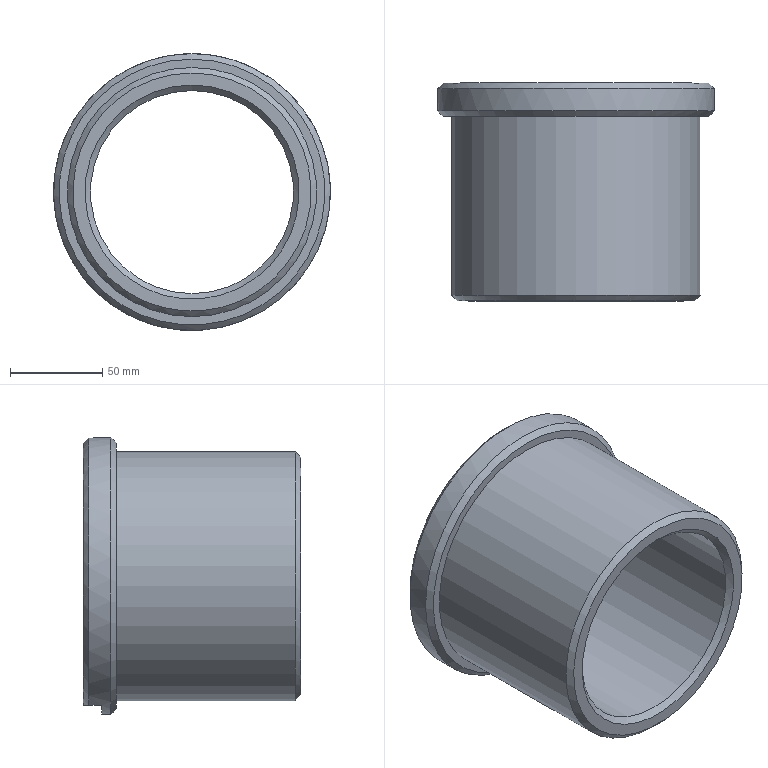Component | NX | BORE_BUSHING | 1 solid | 13 faces | box 150 x 118 x 150 mm | volume 617263 mm3 | plane 5 | cone 5 | cylinder 3 | commonest cylinder face diameters 135 x1 150 x1 110 x1
STEP:
#1=CARTESIAN_POINT('',(0.,0.,0.));
#2=DIRECTION('',(0.,0.,1.));
#3=DIRECTION('',(1.,0.,0.));
#4=AXIS2_PLACEMENT_3D('',#1,#2,#3);
#5=CARTESIAN_POINT('',(0.,42.5,208.));
#6=VERTEX_POINT('',#5);
#7=CARTESIAN_POINT('',(0.,42.5,150.));
#8=DIRECTION('',(0.,1.,0.));
#9=DIRECTION('',(0.,0.,1.));
#10=AXIS2_PLACEMENT_3D('',#7,#8,#9);
#11=CIRCLE('',#10,58.);
#12=CARTESIAN_POINT('',(0.,42.5,150.));
#13=DIRECTION('',(0.,-1.,0.));
#14=DIRECTION('',(0.,0.,1.));
#15=AXIS2_PLACEMENT_3D('',#12,#13,#14);
#16=PLANE('',#15);
#17=CARTESIAN_POINT('',(58.,0.));
#18=CARTESIAN_POINT('',(58.,-100.459));
#19=CARTESIAN_POINT('',(-29.,-50.229));
#20=CARTESIAN_POINT('',(-116.,-0.));
#21=CARTESIAN_POINT('',(-29.,50.229));
#22=CARTESIAN_POINT('',(58.,100.459));
#23=CARTESIAN_POINT('',(58.,0.));
#24=(BOUNDED_CURVE()B_SPLINE_CURVE(2,(#17,#18,#19,#20,#21,#22,#23),.UNSPECIFIED.,.T.,.F.)B_SPLINE_CURVE_WITH_KNOTS((1,2,2,2,2,1),(-2.094,0.,2.094,4.189,6.283,8.378),.UNSPECIFIED.)CURVE()GEOMETRIC_REPRESENTATION_ITEM()RATIONAL_B_SPLINE_CURVE((1.,0.5,1.,0.5,1.,0.5,1.))REPRESENTATION_ITEM(''));
#25=(GEOMETRIC_REPRESENTATION_CONTEXT(2)PARAMETRIC_REPRESENTATION_CONTEXT()REPRESENTATION_CONTEXT('',''));
#26=DEFINITIONAL_REPRESENTATION('',(#24),#25);
#27=PCURVE('',#16,#26);
#28=CARTESIAN_POINT('',(0.,45.5,150.));
#29=DIRECTION('',(0.,-1.,0.));
#30=DIRECTION('',(0.,0.,1.));
#31=AXIS2_PLACEMENT_3D('',#28,#29,#30);
#32=CONICAL_SURFACE('',#31,55.,0.7854);
#33=CARTESIAN_POINT('',(6.283,3.));
#34=DIRECTION('',(-1.,0.));
#35=VECTOR('',#34,1.);
#36=LINE('',#33,#35);
#37=(GEOMETRIC_REPRESENTATION_CONTEXT(2)PARAMETRIC_REPRESENTATION_CONTEXT()REPRESENTATION_CONTEXT('',''));
#38=DEFINITIONAL_REPRESENTATION('',(#36),#37);
#39=PCURVE('',#32,#38);
#40=SURFACE_CURVE('',#11,(#27,#39),.PCURVE_S1.);
#41=EDGE_CURVE('',#6,#6,#40,.T.);
#42=ORIENTED_EDGE('',*,*,#41,.T.);
#43=EDGE_LOOP('',(#42));
#44=FACE_BOUND('',#43,.T.);
#45=CARTESIAN_POINT('',(0.,42.5,214.5));
#46=VERTEX_POINT('',#45);
#47=CARTESIAN_POINT('',(0.,42.5,150.));
#48=DIRECTION('',(0.,-1.,0.));
#49=DIRECTION('',(0.,0.,1.));
#50=AXIS2_PLACEMENT_3D('',#47,#48,#49);
#51=CIRCLE('',#50,64.5);
#52=CARTESIAN_POINT('',(0.,0.));
#53=DIRECTION('',(1.,0.));
#54=AXIS2_PLACEMENT_2D('',#52,#53);
#55=CIRCLE('',#54,64.5);
#56=(GEOMETRIC_REPRESENTATION_CONTEXT(2)PARAMETRIC_REPRESENTATION_CONTEXT()REPRESENTATION_CONTEXT('',''));
#57=DEFINITIONAL_REPRESENTATION('',(#55),#56);
#58=PCURVE('',#16,#57);
#59=CARTESIAN_POINT('',(0.,45.5,150.));
#60=DIRECTION('',(0.,1.,0.));
#61=DIRECTION('',(0.,0.,-1.));
#62=AXIS2_PLACEMENT_3D('',#59,#60,#61);
#63=CONICAL_SURFACE('',#62,67.5,0.7854);
#64=CARTESIAN_POINT('',(9.425,-3.));
#65=DIRECTION('',(-1.,0.));
#66=VECTOR('',#65,1.);
#67=LINE('',#64,#66);
#68=(GEOMETRIC_REPRESENTATION_CONTEXT(2)PARAMETRIC_REPRESENTATION_CONTEXT()REPRESENTATION_CONTEXT('',''));
#69=DEFINITIONAL_REPRESENTATION('',(#67),#68);
#70=PCURVE('',#63,#69);
#71=SURFACE_CURVE('',#51,(#58,#70),.PCURVE_S1.);
#72=EDGE_CURVE('',#46,#46,#71,.T.);
#73=ORIENTED_EDGE('',*,*,#72,.T.);
#74=EDGE_LOOP('',(#73));
#75=FACE_BOUND('',#74,.T.);
#76=ADVANCED_FACE('',(#44,#75),#16,.T.);
#77=CARTESIAN_POINT('',(0.,45.5,217.5));
#78=VERTEX_POINT('',#77);
#79=CARTESIAN_POINT('',(0.,45.5,150.));
#80=DIRECTION('',(0.,1.,0.));
#81=DIRECTION('',(0.,0.,1.));
#82=AXIS2_PLACEMENT_3D('',#79,#80,#81);
#83=CIRCLE('',#82,67.5);
#84=CARTESIAN_POINT('',(0.,42.5,150.));
#85=DIRECTION('',(0.,1.,0.));
#86=DIRECTION('',(0.,0.,-1.));
#87=AXIS2_PLACEMENT_3D('',#84,#85,#86);
#88=CYLINDRICAL_SURFACE('',#87,67.5);
#89=CARTESIAN_POINT('',(3.142,3.));
#90=DIRECTION('',(1.,0.));
#91=VECTOR('',#90,1.);
#92=LINE('',#89,#91);
#93=(GEOMETRIC_REPRESENTATION_CONTEXT(2)PARAMETRIC_REPRESENTATION_CONTEXT()REPRESENTATION_CONTEXT('',''));
#94=DEFINITIONAL_REPRESENTATION('',(#92),#93);
#95=PCURVE('',#88,#94);
#96=CARTESIAN_POINT('',(3.142,0.));
#97=DIRECTION('',(1.,0.));
#98=VECTOR('',#97,1.);
#99=LINE('',#96,#98);
#100=(GEOMETRIC_REPRESENTATION_CONTEXT(2)PARAMETRIC_REPRESENTATION_CONTEXT()REPRESENTATION_CONTEXT('',''));
#101=DEFINITIONAL_REPRESENTATION('',(#99),#100);
#102=PCURVE('',#63,#101);
#103=SURFACE_CURVE('',#83,(#95,#102),.PCURVE_S1.);
#104=EDGE_CURVE('',#78,#78,#103,.T.);
#105=ORIENTED_EDGE('',*,*,#104,.T.);
#106=CARTESIAN_POINT('',(0.,142.5,217.5));
#107=VERTEX_POINT('',#106);
#108=CARTESIAN_POINT('',(-0.,45.5,217.5));
#109=CARTESIAN_POINT('',(-0.,142.5,217.5));
#110=B_SPLINE_CURVE_WITH_KNOTS('',1,(#108,#109),.UNSPECIFIED.,.F.,.F.,(2,2),(3.,100.),.PIECEWISE_BEZIER_KNOTS.);
#111=CARTESIAN_POINT('',(9.425,0.));
#112=DIRECTION('',(0.,1.));
#113=VECTOR('',#112,1.);
#114=LINE('',#111,#113);
#115=(GEOMETRIC_REPRESENTATION_CONTEXT(2)PARAMETRIC_REPRESENTATION_CONTEXT()REPRESENTATION_CONTEXT('',''));
#116=DEFINITIONAL_REPRESENTATION('',(#114),#115);
#117=PCURVE('',#88,#116);
#118=CARTESIAN_POINT('',(3.142,0.));
#119=DIRECTION('',(0.,1.));
#120=VECTOR('',#119,1.);
#121=LINE('',#118,#120);
#122=(GEOMETRIC_REPRESENTATION_CONTEXT(2)PARAMETRIC_REPRESENTATION_CONTEXT()REPRESENTATION_CONTEXT('',''));
#123=DEFINITIONAL_REPRESENTATION('',(#121),#122);
#124=PCURVE('',#88,#123);
#125=SEAM_CURVE('',#110,(#117,#124),.PCURVE_S1.);
#126=EDGE_CURVE('',#78,#107,#125,.T.);
#127=ORIENTED_EDGE('',*,*,#126,.T.);
#128=CARTESIAN_POINT('',(0.,142.5,150.));
#129=DIRECTION('',(0.,1.,0.));
#130=DIRECTION('',(0.,0.,1.));
#131=AXIS2_PLACEMENT_3D('',#128,#129,#130);
#132=CIRCLE('',#131,67.5);
#133=CARTESIAN_POINT('',(3.142,100.));
#134=DIRECTION('',(1.,0.));
#135=VECTOR('',#134,1.);
#136=LINE('',#133,#135);
#137=(GEOMETRIC_REPRESENTATION_CONTEXT(2)PARAMETRIC_REPRESENTATION_CONTEXT()REPRESENTATION_CONTEXT('',''));
#138=DEFINITIONAL_REPRESENTATION('',(#136),#137);
#139=PCURVE('',#88,#138);
#140=CARTESIAN_POINT('',(0.,142.5,150.));
#141=DIRECTION('',(0.,-1.,0.));
#142=DIRECTION('',(0.,0.,1.));
#143=AXIS2_PLACEMENT_3D('',#140,#141,#142);
#144=PLANE('',#143);
#145=CARTESIAN_POINT('',(67.5,0.));
#146=CARTESIAN_POINT('',(67.5,-116.913));
#147=CARTESIAN_POINT('',(-33.75,-58.457));
#148=CARTESIAN_POINT('',(-135.,-0.));
#149=CARTESIAN_POINT('',(-33.75,58.457));
#150=CARTESIAN_POINT('',(67.5,116.913));
#151=CARTESIAN_POINT('',(67.5,0.));
#152=(BOUNDED_CURVE()B_SPLINE_CURVE(2,(#145,#146,#147,#148,#149,#150,#151),.UNSPECIFIED.,.T.,.F.)B_SPLINE_CURVE_WITH_KNOTS((1,2,2,2,2,1),(-2.094,0.,2.094,4.189,6.283,8.378),.UNSPECIFIED.)CURVE()GEOMETRIC_REPRESENTATION_ITEM()RATIONAL_B_SPLINE_CURVE((1.,0.5,1.,0.5,1.,0.5,1.))REPRESENTATION_ITEM(''));
#153=(GEOMETRIC_REPRESENTATION_CONTEXT(2)PARAMETRIC_REPRESENTATION_CONTEXT()REPRESENTATION_CONTEXT('',''));
#154=DEFINITIONAL_REPRESENTATION('',(#152),#153);
#155=PCURVE('',#144,#154);
#156=SURFACE_CURVE('',#132,(#139,#155),.PCURVE_S1.);
#157=EDGE_CURVE('',#107,#107,#156,.T.);
#158=ORIENTED_EDGE('',*,*,#157,.F.);
#159=ORIENTED_EDGE('',*,*,#126,.F.);
#160=EDGE_LOOP('',(#105,#127,#158,#159));
#161=FACE_BOUND('',#160,.T.);
#162=ADVANCED_FACE('',(#161),#88,.T.);
#163=CARTESIAN_POINT('',(0.,160.5,92.));
#164=VERTEX_POINT('',#163);
#165=CARTESIAN_POINT('',(0.,160.5,150.));
#166=DIRECTION('',(0.,-1.,0.));
#167=DIRECTION('',(0.,0.,-1.));
#168=AXIS2_PLACEMENT_3D('',#165,#166,#167);
#169=CIRCLE('',#168,58.);
#170=CARTESIAN_POINT('',(0.,160.5,150.));
#171=DIRECTION('',(0.,1.,0.));
#172=DIRECTION('',(0.,0.,-1.));
#173=AXIS2_PLACEMENT_3D('',#170,#171,#172);
#174=PLANE('',#173);
#175=CARTESIAN_POINT('',(58.,0.));
#176=CARTESIAN_POINT('',(58.,-100.459));
#177=CARTESIAN_POINT('',(-29.,-50.229));
#178=CARTESIAN_POINT('',(-116.,-0.));
#179=CARTESIAN_POINT('',(-29.,50.229));
#180=CARTESIAN_POINT('',(58.,100.459));
#181=CARTESIAN_POINT('',(58.,0.));
#182=(BOUNDED_CURVE()B_SPLINE_CURVE(2,(#175,#176,#177,#178,#179,#180,#181),.UNSPECIFIED.,.T.,.F.)B_SPLINE_CURVE_WITH_KNOTS((1,2,2,2,2,1),(-2.094,0.,2.094,4.189,6.283,8.378),.UNSPECIFIED.)CURVE()GEOMETRIC_REPRESENTATION_ITEM()RATIONAL_B_SPLINE_CURVE((1.,0.5,1.,0.5,1.,0.5,1.))REPRESENTATION_ITEM(''));
#183=(GEOMETRIC_REPRESENTATION_CONTEXT(2)PARAMETRIC_REPRESENTATION_CONTEXT()REPRESENTATION_CONTEXT('',''));
#184=DEFINITIONAL_REPRESENTATION('',(#182),#183);
#185=PCURVE('',#174,#184);
#186=CARTESIAN_POINT('',(0.,160.5,150.));
#187=DIRECTION('',(0.,1.,0.));
#188=DIRECTION('',(0.,0.,-1.));
#189=AXIS2_PLACEMENT_3D('',#186,#187,#188);
#190=CONICAL_SURFACE('',#189,58.,0.7854);
#191=CARTESIAN_POINT('',(6.283,0.));
#192=DIRECTION('',(-1.,0.));
#193=VECTOR('',#192,1.);
#194=LINE('',#191,#193);
#195=(GEOMETRIC_REPRESENTATION_CONTEXT(2)PARAMETRIC_REPRESENTATION_CONTEXT()REPRESENTATION_CONTEXT('',''));
#196=DEFINITIONAL_REPRESENTATION('',(#194),#195);
#197=PCURVE('',#190,#196);
#198=SURFACE_CURVE('',#169,(#185,#197),.PCURVE_S1.);
#199=EDGE_CURVE('',#164,#164,#198,.T.);
#200=ORIENTED_EDGE('',*,*,#199,.T.);
#201=EDGE_LOOP('',(#200));
#202=FACE_BOUND('',#201,.T.);
#203=CARTESIAN_POINT('',(-16.852,160.5,80.));
#204=VERTEX_POINT('',#203);
#205=CARTESIAN_POINT('',(16.852,160.5,80.));
#206=VERTEX_POINT('',#205);
#207=CARTESIAN_POINT('',(-76.,160.5,80.));
#208=DIRECTION('',(1.,0.,-0.));
#209=VECTOR('',#208,1.);
#210=LINE('',#207,#209);
#211=CARTESIAN_POINT('',(70.,76.));
#212=DIRECTION('',(0.,-1.));
#213=VECTOR('',#212,1.);
#214=LINE('',#211,#213);
#215=(GEOMETRIC_REPRESENTATION_CONTEXT(2)PARAMETRIC_REPRESENTATION_CONTEXT()REPRESENTATION_CONTEXT('',''));
#216=DEFINITIONAL_REPRESENTATION('',(#214),#215);
#217=PCURVE('',#174,#216);
#218=CARTESIAN_POINT('',(-76.,150.5,80.));
#219=DIRECTION('',(0.,0.,1.));
#220=DIRECTION('',(1.,0.,-0.));
#221=AXIS2_PLACEMENT_3D('',#218,#219,#220);
#222=PLANE('',#221);
#223=CARTESIAN_POINT('',(0.,10.));
#224=DIRECTION('',(1.,0.));
#225=VECTOR('',#224,1.);
#226=LINE('',#223,#225);
#227=(GEOMETRIC_REPRESENTATION_CONTEXT(2)PARAMETRIC_REPRESENTATION_CONTEXT()REPRESENTATION_CONTEXT('',''));
#228=DEFINITIONAL_REPRESENTATION('',(#226),#227);
#229=PCURVE('',#222,#228);
#230=SURFACE_CURVE('',#210,(#217,#229),.PCURVE_S1.);
#231=EDGE_CURVE('',#204,#206,#230,.T.);
#232=ORIENTED_EDGE('',*,*,#231,.F.);
#233=CARTESIAN_POINT('',(0.,160.5,150.));
#234=DIRECTION('',(0.,1.,0.));
#235=DIRECTION('',(0.,0.,-1.));
#236=AXIS2_PLACEMENT_3D('',#233,#234,#235);
#237=CIRCLE('',#236,72.);
#238=CARTESIAN_POINT('',(0.,0.));
#239=DIRECTION('',(1.,0.));
#240=AXIS2_PLACEMENT_2D('',#238,#239);
#241=CIRCLE('',#240,72.);
#242=(GEOMETRIC_REPRESENTATION_CONTEXT(2)PARAMETRIC_REPRESENTATION_CONTEXT()REPRESENTATION_CONTEXT('',''));
#243=DEFINITIONAL_REPRESENTATION('',(#241),#242);
#244=PCURVE('',#174,#243);
#245=CARTESIAN_POINT('',(0.,157.5,150.));
#246=DIRECTION('',(0.,-1.,0.));
#247=DIRECTION('',(0.,0.,1.));
#248=AXIS2_PLACEMENT_3D('',#245,#246,#247);
#249=CONICAL_SURFACE('',#248,75.,0.7854);
#250=CARTESIAN_POINT('',(3.142,-3.));
#251=DIRECTION('',(-1.,0.));
#252=VECTOR('',#251,1.);
#253=LINE('',#250,#252);
#254=(GEOMETRIC_REPRESENTATION_CONTEXT(2)PARAMETRIC_REPRESENTATION_CONTEXT()REPRESENTATION_CONTEXT('',''));
#255=DEFINITIONAL_REPRESENTATION('',(#253),#254);
#256=PCURVE('',#249,#255);
#257=SURFACE_CURVE('',#237,(#244,#256),.PCURVE_S1.);
#258=EDGE_CURVE('',#204,#206,#257,.T.);
#259=ORIENTED_EDGE('',*,*,#258,.T.);
#260=EDGE_LOOP('',(#232,#259));
#261=FACE_BOUND('',#260,.T.);
#262=ADVANCED_FACE('',(#202,#261),#174,.T.);
#263=CARTESIAN_POINT('',(0.,142.5,222.));
#264=VERTEX_POINT('',#263);
#265=CARTESIAN_POINT('',(0.,142.5,150.));
#266=DIRECTION('',(0.,-1.,0.));
#267=DIRECTION('',(0.,0.,1.));
#268=AXIS2_PLACEMENT_3D('',#265,#266,#267);
#269=CIRCLE('',#268,72.);
#270=CARTESIAN_POINT('',(0.,0.));
#271=DIRECTION('',(1.,0.));
#272=AXIS2_PLACEMENT_2D('',#270,#271);
#273=CIRCLE('',#272,72.);
#274=(GEOMETRIC_REPRESENTATION_CONTEXT(2)PARAMETRIC_REPRESENTATION_CONTEXT()REPRESENTATION_CONTEXT('',''));
#275=DEFINITIONAL_REPRESENTATION('',(#273),#274);
#276=PCURVE('',#144,#275);
#277=CARTESIAN_POINT('',(0.,145.5,150.));
#278=DIRECTION('',(0.,1.,0.));
#279=DIRECTION('',(0.,0.,-1.));
#280=AXIS2_PLACEMENT_3D('',#277,#278,#279);
#281=CONICAL_SURFACE('',#280,75.,0.7854);
#282=CARTESIAN_POINT('',(9.425,-3.));
#283=DIRECTION('',(-1.,0.));
#284=VECTOR('',#283,1.);
#285=LINE('',#282,#284);
#286=(GEOMETRIC_REPRESENTATION_CONTEXT(2)PARAMETRIC_REPRESENTATION_CONTEXT()REPRESENTATION_CONTEXT('',''));
#287=DEFINITIONAL_REPRESENTATION('',(#285),#286);
#288=PCURVE('',#281,#287);
#289=SURFACE_CURVE('',#269,(#276,#288),.PCURVE_S1.);
#290=EDGE_CURVE('',#264,#264,#289,.T.);
#291=ORIENTED_EDGE('',*,*,#290,.T.);
#292=EDGE_LOOP('',(#291));
#293=FACE_BOUND('',#292,.T.);
#294=ORIENTED_EDGE('',*,*,#157,.T.);
#295=EDGE_LOOP('',(#294));
#296=FACE_BOUND('',#295,.T.);
#297=ADVANCED_FACE('',(#293,#296),#144,.T.);
#298=CARTESIAN_POINT('',(0.,145.5,225.));
#299=VERTEX_POINT('',#298);
#300=CARTESIAN_POINT('',(26.926,145.5,80.));
#301=VERTEX_POINT('',#300);
#302=CARTESIAN_POINT('',(0.,145.5,150.));
#303=DIRECTION('',(0.,1.,0.));
#304=DIRECTION('',(0.,0.,1.));
#305=AXIS2_PLACEMENT_3D('',#302,#303,#304);
#306=CIRCLE('',#305,75.);
#307=CARTESIAN_POINT('',(0.,142.5,150.));
#308=DIRECTION('',(0.,1.,0.));
#309=DIRECTION('',(0.,0.,-1.));
#310=AXIS2_PLACEMENT_3D('',#307,#308,#309);
#311=CYLINDRICAL_SURFACE('',#310,75.);
#312=CARTESIAN_POINT('',(9.425,3.));
#313=DIRECTION('',(1.,0.));
#314=VECTOR('',#313,1.);
#315=LINE('',#312,#314);
#316=(GEOMETRIC_REPRESENTATION_CONTEXT(2)PARAMETRIC_REPRESENTATION_CONTEXT()REPRESENTATION_CONTEXT('',''));
#317=DEFINITIONAL_REPRESENTATION('',(#315),#316);
#318=PCURVE('',#311,#317);
#319=CARTESIAN_POINT('',(3.142,0.));
#320=DIRECTION('',(1.,0.));
#321=VECTOR('',#320,1.);
#322=LINE('',#319,#321);
#323=(GEOMETRIC_REPRESENTATION_CONTEXT(2)PARAMETRIC_REPRESENTATION_CONTEXT()REPRESENTATION_CONTEXT('',''));
#324=DEFINITIONAL_REPRESENTATION('',(#322),#323);
#325=PCURVE('',#281,#324);
#326=SURFACE_CURVE('',#306,(#318,#325),.PCURVE_S1.);
#327=EDGE_CURVE('',#299,#301,#326,.T.);
#328=ORIENTED_EDGE('',*,*,#327,.T.);
#329=CARTESIAN_POINT('',(26.926,150.5,80.));
#330=VERTEX_POINT('',#329);
#331=CARTESIAN_POINT('',(26.926,145.5,80.));
#332=CARTESIAN_POINT('',(26.926,150.5,80.));
#333=B_SPLINE_CURVE_WITH_KNOTS('',1,(#331,#332),.UNSPECIFIED.,.F.,.F.,(2,2),(3.,8.),.PIECEWISE_BEZIER_KNOTS.);
#334=CARTESIAN_POINT('',(12.199,0.));
#335=DIRECTION('',(0.,1.));
#336=VECTOR('',#335,1.);
#337=LINE('',#334,#336);
#338=(GEOMETRIC_REPRESENTATION_CONTEXT(2)PARAMETRIC_REPRESENTATION_CONTEXT()REPRESENTATION_CONTEXT('',''));
#339=DEFINITIONAL_REPRESENTATION('',(#337),#338);
#340=PCURVE('',#311,#339);
#341=CARTESIAN_POINT('',(5.916,0.));
#342=DIRECTION('',(0.,1.));
#343=VECTOR('',#342,1.);
#344=LINE('',#341,#343);
#345=(GEOMETRIC_REPRESENTATION_CONTEXT(2)PARAMETRIC_REPRESENTATION_CONTEXT()REPRESENTATION_CONTEXT('',''));
#346=DEFINITIONAL_REPRESENTATION('',(#344),#345);
#347=PCURVE('',#311,#346);
#348=SEAM_CURVE('',#333,(#340,#347),.PCURVE_S1.);
#349=EDGE_CURVE('',#301,#330,#348,.T.);
#350=ORIENTED_EDGE('',*,*,#349,.T.);
#351=CARTESIAN_POINT('',(26.926,157.5,80.));
#352=VERTEX_POINT('',#351);
#353=CARTESIAN_POINT('',(26.926,142.5,80.));
#354=DIRECTION('',(0.,-1.,0.));
#355=VECTOR('',#354,1.);
#356=LINE('',#353,#355);
#357=CARTESIAN_POINT('',(12.199,0.));
#358=DIRECTION('',(0.,-1.));
#359=VECTOR('',#358,1.);
#360=LINE('',#357,#359);
#361=(GEOMETRIC_REPRESENTATION_CONTEXT(2)PARAMETRIC_REPRESENTATION_CONTEXT()REPRESENTATION_CONTEXT('',''));
#362=DEFINITIONAL_REPRESENTATION('',(#360),#361);
#363=PCURVE('',#311,#362);
#364=CARTESIAN_POINT('',(102.926,-8.));
#365=DIRECTION('',(0.,-1.));
#366=VECTOR('',#365,1.);
#367=LINE('',#364,#366);
#368=(GEOMETRIC_REPRESENTATION_CONTEXT(2)PARAMETRIC_REPRESENTATION_CONTEXT()REPRESENTATION_CONTEXT('',''));
#369=DEFINITIONAL_REPRESENTATION('',(#367),#368);
#370=PCURVE('',#222,#369);
#371=SURFACE_CURVE('',#356,(#363,#370),.PCURVE_S1.);
#372=EDGE_CURVE('',#352,#330,#371,.T.);
#373=ORIENTED_EDGE('',*,*,#372,.F.);
#374=CARTESIAN_POINT('',(-26.926,157.5,80.));
#375=VERTEX_POINT('',#374);
#376=CARTESIAN_POINT('',(0.,157.5,150.));
#377=DIRECTION('',(0.,-1.,0.));
#378=DIRECTION('',(0.,0.,-1.));
#379=AXIS2_PLACEMENT_3D('',#376,#377,#378);
#380=CIRCLE('',#379,75.);
#381=CARTESIAN_POINT('',(12.566,15.));
#382=DIRECTION('',(-1.,0.));
#383=VECTOR('',#382,1.);
#384=LINE('',#381,#383);
#385=(GEOMETRIC_REPRESENTATION_CONTEXT(2)PARAMETRIC_REPRESENTATION_CONTEXT()REPRESENTATION_CONTEXT('',''));
#386=DEFINITIONAL_REPRESENTATION('',(#384),#385);
#387=PCURVE('',#311,#386);
#388=CARTESIAN_POINT('',(-3.142,0.));
#389=DIRECTION('',(1.,0.));
#390=VECTOR('',#389,1.);
#391=LINE('',#388,#390);
#392=(GEOMETRIC_REPRESENTATION_CONTEXT(2)PARAMETRIC_REPRESENTATION_CONTEXT()REPRESENTATION_CONTEXT('',''));
#393=DEFINITIONAL_REPRESENTATION('',(#391),#392);
#394=PCURVE('',#249,#393);
#395=SURFACE_CURVE('',#380,(#387,#394),.PCURVE_S1.);
#396=EDGE_CURVE('',#352,#375,#395,.T.);
#397=ORIENTED_EDGE('',*,*,#396,.T.);
#398=CARTESIAN_POINT('',(-26.926,150.5,80.));
#399=VERTEX_POINT('',#398);
#400=CARTESIAN_POINT('',(-26.926,142.5,80.));
#401=DIRECTION('',(0.,1.,0.));
#402=VECTOR('',#401,1.);
#403=LINE('',#400,#402);
#404=CARTESIAN_POINT('',(6.65,0.));
#405=DIRECTION('',(0.,1.));
#406=VECTOR('',#405,1.);
#407=LINE('',#404,#406);
#408=(GEOMETRIC_REPRESENTATION_CONTEXT(2)PARAMETRIC_REPRESENTATION_CONTEXT()REPRESENTATION_CONTEXT('',''));
#409=DEFINITIONAL_REPRESENTATION('',(#407),#408);
#410=PCURVE('',#311,#409);
#411=CARTESIAN_POINT('',(49.074,-8.));
#412=DIRECTION('',(0.,1.));
#413=VECTOR('',#412,1.);
#414=LINE('',#411,#413);
#415=(GEOMETRIC_REPRESENTATION_CONTEXT(2)PARAMETRIC_REPRESENTATION_CONTEXT()REPRESENTATION_CONTEXT('',''));
#416=DEFINITIONAL_REPRESENTATION('',(#414),#415);
#417=PCURVE('',#222,#416);
#418=SURFACE_CURVE('',#403,(#410,#417),.PCURVE_S1.);
#419=EDGE_CURVE('',#399,#375,#418,.T.);
#420=ORIENTED_EDGE('',*,*,#419,.F.);
#421=CARTESIAN_POINT('',(0.,150.5,150.));
#422=DIRECTION('',(0.,-1.,0.));
#423=DIRECTION('',(0.,0.,-1.));
#424=AXIS2_PLACEMENT_3D('',#421,#422,#423);
#425=CIRCLE('',#424,75.);
#426=CARTESIAN_POINT('',(12.566,8.));
#427=DIRECTION('',(-1.,0.));
#428=VECTOR('',#427,1.);
#429=LINE('',#426,#428);
#430=(GEOMETRIC_REPRESENTATION_CONTEXT(2)PARAMETRIC_REPRESENTATION_CONTEXT()REPRESENTATION_CONTEXT('',''));
#431=DEFINITIONAL_REPRESENTATION('',(#429),#430);
#432=PCURVE('',#311,#431);
#433=CARTESIAN_POINT('',(0.,150.5,150.));
#434=DIRECTION('',(0.,1.,0.));
#435=DIRECTION('',(0.,0.,-1.));
#436=AXIS2_PLACEMENT_3D('',#433,#434,#435);
#437=PLANE('',#436);
#438=CARTESIAN_POINT('',(75.,0.));
#439=CARTESIAN_POINT('',(75.,-129.904));
#440=CARTESIAN_POINT('',(-37.5,-64.952));
#441=CARTESIAN_POINT('',(-150.,-0.));
#442=CARTESIAN_POINT('',(-37.5,64.952));
#443=CARTESIAN_POINT('',(75.,129.904));
#444=CARTESIAN_POINT('',(75.,0.));
#445=(BOUNDED_CURVE()B_SPLINE_CURVE(2,(#438,#439,#440,#441,#442,#443,#444),.UNSPECIFIED.,.T.,.F.)B_SPLINE_CURVE_WITH_KNOTS((1,2,2,2,2,1),(-2.094,0.,2.094,4.189,6.283,8.378),.UNSPECIFIED.)CURVE()GEOMETRIC_REPRESENTATION_ITEM()RATIONAL_B_SPLINE_CURVE((1.,0.5,1.,0.5,1.,0.5,1.))REPRESENTATION_ITEM(''));
#446=(GEOMETRIC_REPRESENTATION_CONTEXT(2)PARAMETRIC_REPRESENTATION_CONTEXT()REPRESENTATION_CONTEXT('',''));
#447=DEFINITIONAL_REPRESENTATION('',(#445),#446);
#448=PCURVE('',#437,#447);
#449=SURFACE_CURVE('',#425,(#432,#448),.PCURVE_S1.);
#450=EDGE_CURVE('',#399,#330,#449,.T.);
#451=ORIENTED_EDGE('',*,*,#450,.T.);
#452=ORIENTED_EDGE('',*,*,#349,.F.);
#453=CARTESIAN_POINT('',(0.,145.5,150.));
#454=DIRECTION('',(0.,1.,0.));
#455=DIRECTION('',(0.,0.,1.));
#456=AXIS2_PLACEMENT_3D('',#453,#454,#455);
#457=CIRCLE('',#456,75.);
#458=CARTESIAN_POINT('',(3.142,3.));
#459=DIRECTION('',(1.,0.));
#460=VECTOR('',#459,1.);
#461=LINE('',#458,#460);
#462=(GEOMETRIC_REPRESENTATION_CONTEXT(2)PARAMETRIC_REPRESENTATION_CONTEXT()REPRESENTATION_CONTEXT('',''));
#463=DEFINITIONAL_REPRESENTATION('',(#461),#462);
#464=PCURVE('',#311,#463);
#465=CARTESIAN_POINT('',(3.142,0.));
#466=DIRECTION('',(1.,0.));
#467=VECTOR('',#466,1.);
#468=LINE('',#465,#467);
#469=(GEOMETRIC_REPRESENTATION_CONTEXT(2)PARAMETRIC_REPRESENTATION_CONTEXT()REPRESENTATION_CONTEXT('',''));
#470=DEFINITIONAL_REPRESENTATION('',(#468),#469);
#471=PCURVE('',#281,#470);
#472=SURFACE_CURVE('',#457,(#464,#471),.PCURVE_S1.);
#473=EDGE_CURVE('',#301,#299,#472,.T.);
#474=ORIENTED_EDGE('',*,*,#473,.T.);
#475=EDGE_LOOP('',(#328,#350,#373,#397,#420,#451,#452,#474));
#476=FACE_BOUND('',#475,.T.);
#477=ADVANCED_FACE('',(#476),#311,.T.);
#478=CARTESIAN_POINT('',(0.,45.5,205.));
#479=VERTEX_POINT('',#478);
#480=CARTESIAN_POINT('',(0.,45.5,150.));
#481=DIRECTION('',(0.,-1.,0.));
#482=DIRECTION('',(0.,0.,1.));
#483=AXIS2_PLACEMENT_3D('',#480,#481,#482);
#484=CIRCLE('',#483,55.);
#485=CARTESIAN_POINT('',(0.,160.5,150.));
#486=DIRECTION('',(0.,-1.,0.));
#487=DIRECTION('',(0.,0.,1.));
#488=AXIS2_PLACEMENT_3D('',#485,#486,#487);
#489=CYLINDRICAL_SURFACE('',#488,55.);
#490=CARTESIAN_POINT('',(0.,115.));
#491=DIRECTION('',(1.,0.));
#492=VECTOR('',#491,1.);
#493=LINE('',#490,#492);
#494=(GEOMETRIC_REPRESENTATION_CONTEXT(2)PARAMETRIC_REPRESENTATION_CONTEXT()REPRESENTATION_CONTEXT('',''));
#495=DEFINITIONAL_REPRESENTATION('',(#493),#494);
#496=PCURVE('',#489,#495);
#497=CARTESIAN_POINT('',(0.,0.));
#498=DIRECTION('',(1.,0.));
#499=VECTOR('',#498,1.);
#500=LINE('',#497,#499);
#501=(GEOMETRIC_REPRESENTATION_CONTEXT(2)PARAMETRIC_REPRESENTATION_CONTEXT()REPRESENTATION_CONTEXT('',''));
#502=DEFINITIONAL_REPRESENTATION('',(#500),#501);
#503=PCURVE('',#32,#502);
#504=SURFACE_CURVE('',#484,(#496,#503),.PCURVE_S1.);
#505=EDGE_CURVE('',#479,#479,#504,.T.);
#506=ORIENTED_EDGE('',*,*,#505,.F.);
#507=CARTESIAN_POINT('',(0.,157.5,205.));
#508=VERTEX_POINT('',#507);
#509=CARTESIAN_POINT('',(0.,157.5,205.));
#510=CARTESIAN_POINT('',(0.,45.5,205.));
#511=B_SPLINE_CURVE_WITH_KNOTS('',1,(#509,#510),.UNSPECIFIED.,.F.,.F.,(2,2),(3.,115.),.PIECEWISE_BEZIER_KNOTS.);
#512=CARTESIAN_POINT('',(0.,0.));
#513=DIRECTION('',(0.,1.));
#514=VECTOR('',#513,1.);
#515=LINE('',#512,#514);
#516=(GEOMETRIC_REPRESENTATION_CONTEXT(2)PARAMETRIC_REPRESENTATION_CONTEXT()REPRESENTATION_CONTEXT('',''));
#517=DEFINITIONAL_REPRESENTATION('',(#515),#516);
#518=PCURVE('',#489,#517);
#519=CARTESIAN_POINT('',(6.283,0.));
#520=DIRECTION('',(0.,1.));
#521=VECTOR('',#520,1.);
#522=LINE('',#519,#521);
#523=(GEOMETRIC_REPRESENTATION_CONTEXT(2)PARAMETRIC_REPRESENTATION_CONTEXT()REPRESENTATION_CONTEXT('',''));
#524=DEFINITIONAL_REPRESENTATION('',(#522),#523);
#525=PCURVE('',#489,#524);
#526=SEAM_CURVE('',#511,(#518,#525),.PCURVE_S1.);
#527=EDGE_CURVE('',#508,#479,#526,.T.);
#528=ORIENTED_EDGE('',*,*,#527,.F.);
#529=CARTESIAN_POINT('',(0.,157.5,95.));
#530=VERTEX_POINT('',#529);
#531=CARTESIAN_POINT('',(0.,157.5,150.));
#532=DIRECTION('',(0.,1.,0.));
#533=DIRECTION('',(0.,0.,-1.));
#534=AXIS2_PLACEMENT_3D('',#531,#532,#533);
#535=CIRCLE('',#534,55.);
#536=CARTESIAN_POINT('',(3.142,3.));
#537=DIRECTION('',(-1.,0.));
#538=VECTOR('',#537,1.);
#539=LINE('',#536,#538);
#540=(GEOMETRIC_REPRESENTATION_CONTEXT(2)PARAMETRIC_REPRESENTATION_CONTEXT()REPRESENTATION_CONTEXT('',''));
#541=DEFINITIONAL_REPRESENTATION('',(#539),#540);
#542=PCURVE('',#489,#541);
#543=CARTESIAN_POINT('',(0.,-3.));
#544=DIRECTION('',(1.,0.));
#545=VECTOR('',#544,1.);
#546=LINE('',#543,#545);
#547=(GEOMETRIC_REPRESENTATION_CONTEXT(2)PARAMETRIC_REPRESENTATION_CONTEXT()REPRESENTATION_CONTEXT('',''));
#548=DEFINITIONAL_REPRESENTATION('',(#546),#547);
#549=PCURVE('',#190,#548);
#550=SURFACE_CURVE('',#535,(#542,#549),.PCURVE_S1.);
#551=EDGE_CURVE('',#530,#508,#550,.T.);
#552=ORIENTED_EDGE('',*,*,#551,.F.);
#553=CARTESIAN_POINT('',(0.,157.5,150.));
#554=DIRECTION('',(0.,1.,0.));
#555=DIRECTION('',(0.,0.,-1.));
#556=AXIS2_PLACEMENT_3D('',#553,#554,#555);
#557=CIRCLE('',#556,55.);
#558=CARTESIAN_POINT('',(9.425,3.));
#559=DIRECTION('',(-1.,0.));
#560=VECTOR('',#559,1.);
#561=LINE('',#558,#560);
#562=(GEOMETRIC_REPRESENTATION_CONTEXT(2)PARAMETRIC_REPRESENTATION_CONTEXT()REPRESENTATION_CONTEXT('',''));
#563=DEFINITIONAL_REPRESENTATION('',(#561),#562);
#564=PCURVE('',#489,#563);
#565=CARTESIAN_POINT('',(0.,-3.));
#566=DIRECTION('',(1.,0.));
#567=VECTOR('',#566,1.);
#568=LINE('',#565,#567);
#569=(GEOMETRIC_REPRESENTATION_CONTEXT(2)PARAMETRIC_REPRESENTATION_CONTEXT()REPRESENTATION_CONTEXT('',''));
#570=DEFINITIONAL_REPRESENTATION('',(#568),#569);
#571=PCURVE('',#190,#570);
#572=SURFACE_CURVE('',#557,(#564,#571),.PCURVE_S1.);
#573=EDGE_CURVE('',#508,#530,#572,.T.);
#574=ORIENTED_EDGE('',*,*,#573,.F.);
#575=ORIENTED_EDGE('',*,*,#527,.T.);
#576=EDGE_LOOP('',(#506,#528,#552,#574,#575));
#577=FACE_BOUND('',#576,.F.);
#578=ADVANCED_FACE('',(#577),#489,.F.);
#579=ORIENTED_EDGE('',*,*,#419,.T.);
#580=CARTESIAN_POINT('',(-26.926,157.5,80.));
#581=CARTESIAN_POINT('',(-23.623,158.686,80.));
#582=CARTESIAN_POINT('',(-20.27,159.7,80.));
#583=CARTESIAN_POINT('',(-16.852,160.5,80.));
#584=B_SPLINE_CURVE_WITH_KNOTS('',3,(#580,#581,#582,#583),.UNSPECIFIED.,.F.,.F.,(4,4),(0.,1.),.PIECEWISE_BEZIER_KNOTS.);
#585=CARTESIAN_POINT('',(49.074,7.));
#586=CARTESIAN_POINT('',(52.377,8.186));
#587=CARTESIAN_POINT('',(55.73,9.2));
#588=CARTESIAN_POINT('',(59.148,10.));
#589=B_SPLINE_CURVE_WITH_KNOTS('',3,(#585,#586,#587,#588),.UNSPECIFIED.,.F.,.F.,(4,4),(0.,1.),.PIECEWISE_BEZIER_KNOTS.);
#590=(GEOMETRIC_REPRESENTATION_CONTEXT(2)PARAMETRIC_REPRESENTATION_CONTEXT()REPRESENTATION_CONTEXT('',''));
#591=DEFINITIONAL_REPRESENTATION('',(#589),#590);
#592=PCURVE('',#222,#591);
#593=CARTESIAN_POINT('',(2.774,-0.));
#594=CARTESIAN_POINT('',(2.776,-0.05389));
#595=CARTESIAN_POINT('',(2.78,-0.161));
#596=CARTESIAN_POINT('',(2.786,-0.3194));
#597=CARTESIAN_POINT('',(2.791,-0.4757));
#598=CARTESIAN_POINT('',(2.797,-0.6298));
#599=CARTESIAN_POINT('',(2.803,-0.7817));
#600=CARTESIAN_POINT('',(2.809,-0.9313));
#601=CARTESIAN_POINT('',(2.814,-1.079));
#602=CARTESIAN_POINT('',(2.82,-1.224));
#603=CARTESIAN_POINT('',(2.826,-1.367));
#604=CARTESIAN_POINT('',(2.832,-1.507));
#605=CARTESIAN_POINT('',(2.838,-1.645));
#606=CARTESIAN_POINT('',(2.844,-1.781));
#607=CARTESIAN_POINT('',(2.85,-1.914));
#608=CARTESIAN_POINT('',(2.856,-2.045));
#609=CARTESIAN_POINT('',(2.862,-2.173));
#610=CARTESIAN_POINT('',(2.868,-2.299));
#611=CARTESIAN_POINT('',(2.874,-2.422));
#612=CARTESIAN_POINT('',(2.88,-2.543));
#613=CARTESIAN_POINT('',(2.887,-2.661));
#614=CARTESIAN_POINT('',(2.893,-2.777));
#615=CARTESIAN_POINT('',(2.899,-2.89));
#616=CARTESIAN_POINT('',(2.903,-2.964));
#617=CARTESIAN_POINT('',(2.905,-3.));
#618=B_SPLINE_CURVE_WITH_KNOTS('',3,(#593,#594,#595,#596,#597,#598,#599,#600,#601,#602,#603,#604,#605,#606,#607,#608,#609,#610,#611,#612,#613,#614,#615,#616,#617),.UNSPECIFIED.,.F.,.F.,(4,1,1,1,1,1,1,1,1,1,1,1,1,1,1,1,1,1,1,1,1,1,4),(0.,0.04545,0.09091,0.1364,0.1818,0.2273,0.2727,0.3182,0.3636,0.4091,0.4545,0.5,0.5455,0.5909,0.6364,0.6818,0.7273,0.7727,0.8182,0.8636,0.9091,0.9545,1.),.QUASI_UNIFORM_KNOTS.);
#619=(GEOMETRIC_REPRESENTATION_CONTEXT(2)PARAMETRIC_REPRESENTATION_CONTEXT()REPRESENTATION_CONTEXT('',''));
#620=DEFINITIONAL_REPRESENTATION('',(#618),#619);
#621=PCURVE('',#249,#620);
#622=SURFACE_CURVE('',#584,(#592,#621),.PCURVE_S1.);
#623=EDGE_CURVE('',#375,#204,#622,.T.);
#624=ORIENTED_EDGE('',*,*,#623,.T.);
#625=ORIENTED_EDGE('',*,*,#231,.T.);
#626=CARTESIAN_POINT('',(16.852,160.5,80.));
#627=CARTESIAN_POINT('',(20.27,159.7,80.));
#628=CARTESIAN_POINT('',(23.623,158.686,80.));
#629=CARTESIAN_POINT('',(26.926,157.5,80.));
#630=B_SPLINE_CURVE_WITH_KNOTS('',3,(#626,#627,#628,#629),.UNSPECIFIED.,.F.,.F.,(4,4),(0.,1.),.PIECEWISE_BEZIER_KNOTS.);
#631=CARTESIAN_POINT('',(92.852,10.));
#632=CARTESIAN_POINT('',(96.27,9.2));
#633=CARTESIAN_POINT('',(99.623,8.186));
#634=CARTESIAN_POINT('',(102.926,7.));
#635=B_SPLINE_CURVE_WITH_KNOTS('',3,(#631,#632,#633,#634),.UNSPECIFIED.,.F.,.F.,(4,4),(0.,1.),.PIECEWISE_BEZIER_KNOTS.);
#636=(GEOMETRIC_REPRESENTATION_CONTEXT(2)PARAMETRIC_REPRESENTATION_CONTEXT()REPRESENTATION_CONTEXT('',''));
#637=DEFINITIONAL_REPRESENTATION('',(#635),#636);
#638=PCURVE('',#222,#637);
#639=CARTESIAN_POINT('',(-2.905,-3.));
#640=CARTESIAN_POINT('',(-2.903,-2.964));
#641=CARTESIAN_POINT('',(-2.899,-2.89));
#642=CARTESIAN_POINT('',(-2.893,-2.777));
#643=CARTESIAN_POINT('',(-2.887,-2.661));
#644=CARTESIAN_POINT('',(-2.88,-2.543));
#645=CARTESIAN_POINT('',(-2.874,-2.422));
#646=CARTESIAN_POINT('',(-2.868,-2.299));
#647=CARTESIAN_POINT('',(-2.862,-2.173));
#648=CARTESIAN_POINT('',(-2.856,-2.045));
#649=CARTESIAN_POINT('',(-2.85,-1.914));
#650=CARTESIAN_POINT('',(-2.844,-1.781));
#651=CARTESIAN_POINT('',(-2.838,-1.645));
#652=CARTESIAN_POINT('',(-2.832,-1.507));
#653=CARTESIAN_POINT('',(-2.826,-1.367));
#654=CARTESIAN_POINT('',(-2.82,-1.224));
#655=CARTESIAN_POINT('',(-2.814,-1.079));
#656=CARTESIAN_POINT('',(-2.809,-0.9313));
#657=CARTESIAN_POINT('',(-2.803,-0.7817));
#658=CARTESIAN_POINT('',(-2.797,-0.6298));
#659=CARTESIAN_POINT('',(-2.791,-0.4757));
#660=CARTESIAN_POINT('',(-2.786,-0.3194));
#661=CARTESIAN_POINT('',(-2.78,-0.161));
#662=CARTESIAN_POINT('',(-2.776,-0.05389));
#663=CARTESIAN_POINT('',(-2.774,0.));
#664=B_SPLINE_CURVE_WITH_KNOTS('',3,(#639,#640,#641,#642,#643,#644,#645,#646,#647,#648,#649,#650,#651,#652,#653,#654,#655,#656,#657,#658,#659,#660,#661,#662,#663),.UNSPECIFIED.,.F.,.F.,(4,1,1,1,1,1,1,1,1,1,1,1,1,1,1,1,1,1,1,1,1,1,4),(0.,0.04545,0.09091,0.1364,0.1818,0.2273,0.2727,0.3182,0.3636,0.4091,0.4545,0.5,0.5455,0.5909,0.6364,0.6818,0.7273,0.7727,0.8182,0.8636,0.9091,0.9545,1.),.QUASI_UNIFORM_KNOTS.);
#665=(GEOMETRIC_REPRESENTATION_CONTEXT(2)PARAMETRIC_REPRESENTATION_CONTEXT()REPRESENTATION_CONTEXT('',''));
#666=DEFINITIONAL_REPRESENTATION('',(#664),#665);
#667=PCURVE('',#249,#666);
#668=SURFACE_CURVE('',#630,(#638,#667),.PCURVE_S1.);
#669=EDGE_CURVE('',#206,#352,#668,.T.);
#670=ORIENTED_EDGE('',*,*,#669,.T.);
#671=ORIENTED_EDGE('',*,*,#372,.T.);
#672=CARTESIAN_POINT('',(-76.,150.5,80.));
#673=DIRECTION('',(-1.,0.,0.));
#674=VECTOR('',#673,1.);
#675=LINE('',#672,#674);
#676=CARTESIAN_POINT('',(0.,0.));
#677=DIRECTION('',(-1.,0.));
#678=VECTOR('',#677,1.);
#679=LINE('',#676,#678);
#680=(GEOMETRIC_REPRESENTATION_CONTEXT(2)PARAMETRIC_REPRESENTATION_CONTEXT()REPRESENTATION_CONTEXT('',''));
#681=DEFINITIONAL_REPRESENTATION('',(#679),#680);
#682=PCURVE('',#222,#681);
#683=CARTESIAN_POINT('',(70.,76.));
#684=DIRECTION('',(-0.,1.));
#685=VECTOR('',#684,1.);
#686=LINE('',#683,#685);
#687=(GEOMETRIC_REPRESENTATION_CONTEXT(2)PARAMETRIC_REPRESENTATION_CONTEXT()REPRESENTATION_CONTEXT('',''));
#688=DEFINITIONAL_REPRESENTATION('',(#686),#687);
#689=PCURVE('',#437,#688);
#690=SURFACE_CURVE('',#675,(#682,#689),.PCURVE_S1.);
#691=EDGE_CURVE('',#330,#399,#690,.T.);
#692=ORIENTED_EDGE('',*,*,#691,.T.);
#693=EDGE_LOOP('',(#579,#624,#625,#670,#671,#692));
#694=FACE_BOUND('',#693,.T.);
#695=ADVANCED_FACE('',(#694),#222,.F.);
#696=ORIENTED_EDGE('',*,*,#691,.F.);
#697=ORIENTED_EDGE('',*,*,#450,.F.);
#698=EDGE_LOOP('',(#696,#697));
#699=FACE_BOUND('',#698,.T.);
#700=ADVANCED_FACE('',(#699),#437,.T.);
#701=ORIENTED_EDGE('',*,*,#41,.T.);
#702=CARTESIAN_POINT('',(0.,45.5,205.));
#703=CARTESIAN_POINT('',(0.,42.5,208.));
#704=B_SPLINE_CURVE_WITH_KNOTS('',1,(#702,#703),.UNSPECIFIED.,.F.,.F.,(2,2),(0.,4.243),.PIECEWISE_BEZIER_KNOTS.);
#705=CARTESIAN_POINT('',(0.,0.));
#706=DIRECTION('',(0.,1.));
#707=VECTOR('',#706,1.);
#708=LINE('',#705,#707);
#709=(GEOMETRIC_REPRESENTATION_CONTEXT(2)PARAMETRIC_REPRESENTATION_CONTEXT()REPRESENTATION_CONTEXT('',''));
#710=DEFINITIONAL_REPRESENTATION('',(#708),#709);
#711=PCURVE('',#32,#710);
#712=CARTESIAN_POINT('',(6.283,0.));
#713=DIRECTION('',(0.,1.));
#714=VECTOR('',#713,1.);
#715=LINE('',#712,#714);
#716=(GEOMETRIC_REPRESENTATION_CONTEXT(2)PARAMETRIC_REPRESENTATION_CONTEXT()REPRESENTATION_CONTEXT('',''));
#717=DEFINITIONAL_REPRESENTATION('',(#715),#716);
#718=PCURVE('',#32,#717);
#719=SEAM_CURVE('',#704,(#711,#718),.PCURVE_S1.);
#720=EDGE_CURVE('',#479,#6,#719,.T.);
#721=ORIENTED_EDGE('',*,*,#720,.F.);
#722=ORIENTED_EDGE('',*,*,#505,.T.);
#723=ORIENTED_EDGE('',*,*,#720,.T.);
#724=EDGE_LOOP('',(#701,#721,#722,#723));
#725=FACE_BOUND('',#724,.F.);
#726=ADVANCED_FACE('',(#725),#32,.F.);
#727=ORIENTED_EDGE('',*,*,#72,.F.);
#728=CARTESIAN_POINT('',(-0.,42.5,214.5));
#729=CARTESIAN_POINT('',(-0.,45.5,217.5));
#730=B_SPLINE_CURVE_WITH_KNOTS('',1,(#728,#729),.UNSPECIFIED.,.F.,.F.,(2,2),(-4.243,0.),.PIECEWISE_BEZIER_KNOTS.);
#731=CARTESIAN_POINT('',(9.425,0.));
#732=DIRECTION('',(0.,1.));
#733=VECTOR('',#732,1.);
#734=LINE('',#731,#733);
#735=(GEOMETRIC_REPRESENTATION_CONTEXT(2)PARAMETRIC_REPRESENTATION_CONTEXT()REPRESENTATION_CONTEXT('',''));
#736=DEFINITIONAL_REPRESENTATION('',(#734),#735);
#737=PCURVE('',#63,#736);
#738=CARTESIAN_POINT('',(3.142,0.));
#739=DIRECTION('',(0.,1.));
#740=VECTOR('',#739,1.);
#741=LINE('',#738,#740);
#742=(GEOMETRIC_REPRESENTATION_CONTEXT(2)PARAMETRIC_REPRESENTATION_CONTEXT()REPRESENTATION_CONTEXT('',''));
#743=DEFINITIONAL_REPRESENTATION('',(#741),#742);
#744=PCURVE('',#63,#743);
#745=SEAM_CURVE('',#730,(#737,#744),.PCURVE_S1.);
#746=EDGE_CURVE('',#46,#78,#745,.T.);
#747=ORIENTED_EDGE('',*,*,#746,.T.);
#748=ORIENTED_EDGE('',*,*,#104,.F.);
#749=ORIENTED_EDGE('',*,*,#746,.F.);
#750=EDGE_LOOP('',(#727,#747,#748,#749));
#751=FACE_BOUND('',#750,.T.);
#752=ADVANCED_FACE('',(#751),#63,.T.);
#753=ORIENTED_EDGE('',*,*,#290,.F.);
#754=CARTESIAN_POINT('',(-0.,142.5,222.));
#755=CARTESIAN_POINT('',(-0.,145.5,225.));
#756=B_SPLINE_CURVE_WITH_KNOTS('',1,(#754,#755),.UNSPECIFIED.,.F.,.F.,(2,2),(-4.243,0.),.PIECEWISE_BEZIER_KNOTS.);
#757=CARTESIAN_POINT('',(9.425,0.));
#758=DIRECTION('',(0.,1.));
#759=VECTOR('',#758,1.);
#760=LINE('',#757,#759);
#761=(GEOMETRIC_REPRESENTATION_CONTEXT(2)PARAMETRIC_REPRESENTATION_CONTEXT()REPRESENTATION_CONTEXT('',''));
#762=DEFINITIONAL_REPRESENTATION('',(#760),#761);
#763=PCURVE('',#281,#762);
#764=CARTESIAN_POINT('',(3.142,0.));
#765=DIRECTION('',(0.,1.));
#766=VECTOR('',#765,1.);
#767=LINE('',#764,#766);
#768=(GEOMETRIC_REPRESENTATION_CONTEXT(2)PARAMETRIC_REPRESENTATION_CONTEXT()REPRESENTATION_CONTEXT('',''));
#769=DEFINITIONAL_REPRESENTATION('',(#767),#768);
#770=PCURVE('',#281,#769);
#771=SEAM_CURVE('',#756,(#763,#770),.PCURVE_S1.);
#772=EDGE_CURVE('',#264,#299,#771,.T.);
#773=ORIENTED_EDGE('',*,*,#772,.T.);
#774=ORIENTED_EDGE('',*,*,#473,.F.);
#775=ORIENTED_EDGE('',*,*,#327,.F.);
#776=ORIENTED_EDGE('',*,*,#772,.F.);
#777=EDGE_LOOP('',(#753,#773,#774,#775,#776));
#778=FACE_BOUND('',#777,.T.);
#779=ADVANCED_FACE('',(#778),#281,.T.);
#780=ORIENTED_EDGE('',*,*,#573,.T.);
#781=CARTESIAN_POINT('',(0.,157.5,95.));
#782=CARTESIAN_POINT('',(0.,160.5,92.));
#783=B_SPLINE_CURVE_WITH_KNOTS('',1,(#781,#782),.UNSPECIFIED.,.F.,.F.,(2,2),(-4.243,0.),.PIECEWISE_BEZIER_KNOTS.);
#784=CARTESIAN_POINT('',(6.283,0.));
#785=DIRECTION('',(0.,1.));
#786=VECTOR('',#785,1.);
#787=LINE('',#784,#786);
#788=(GEOMETRIC_REPRESENTATION_CONTEXT(2)PARAMETRIC_REPRESENTATION_CONTEXT()REPRESENTATION_CONTEXT('',''));
#789=DEFINITIONAL_REPRESENTATION('',(#787),#788);
#790=PCURVE('',#190,#789);
#791=CARTESIAN_POINT('',(0.,0.));
#792=DIRECTION('',(0.,1.));
#793=VECTOR('',#792,1.);
#794=LINE('',#791,#793);
#795=(GEOMETRIC_REPRESENTATION_CONTEXT(2)PARAMETRIC_REPRESENTATION_CONTEXT()REPRESENTATION_CONTEXT('',''));
#796=DEFINITIONAL_REPRESENTATION('',(#794),#795);
#797=PCURVE('',#190,#796);
#798=SEAM_CURVE('',#783,(#790,#797),.PCURVE_S1.);
#799=EDGE_CURVE('',#530,#164,#798,.T.);
#800=ORIENTED_EDGE('',*,*,#799,.T.);
#801=ORIENTED_EDGE('',*,*,#199,.T.);
#802=ORIENTED_EDGE('',*,*,#799,.F.);
#803=ORIENTED_EDGE('',*,*,#551,.T.);
#804=EDGE_LOOP('',(#780,#800,#801,#802,#803));
#805=FACE_BOUND('',#804,.F.);
#806=ADVANCED_FACE('',(#805),#190,.F.);
#807=ORIENTED_EDGE('',*,*,#669,.F.);
#808=ORIENTED_EDGE('',*,*,#258,.F.);
#809=ORIENTED_EDGE('',*,*,#623,.F.);
#810=ORIENTED_EDGE('',*,*,#396,.F.);
#811=EDGE_LOOP('',(#807,#808,#809,#810));
#812=FACE_BOUND('',#811,.T.);
#813=ADVANCED_FACE('',(#812),#249,.T.);
#814=CLOSED_SHELL('',(#76,#162,#262,#297,#477,#578,#695,#700,#726,#752,#779,#806,#813));
#815=MANIFOLD_SOLID_BREP('',#814);
#816=(LENGTH_UNIT()NAMED_UNIT(*)SI_UNIT(.MILLI.,.METRE.));
#817=UNCERTAINTY_MEASURE_WITH_UNIT(LENGTH_MEASURE(0.00002),#816,'','');
#818=(NAMED_UNIT(*)PLANE_ANGLE_UNIT()SI_UNIT($,.RADIAN.));
#819=(NAMED_UNIT(*)SI_UNIT($,.STERADIAN.)SOLID_ANGLE_UNIT());
#820=(GEOMETRIC_REPRESENTATION_CONTEXT(3)GLOBAL_UNCERTAINTY_ASSIGNED_CONTEXT((#817))GLOBAL_UNIT_ASSIGNED_CONTEXT((#816,#818,#819))REPRESENTATION_CONTEXT('',''));
#821=ADVANCED_BREP_SHAPE_REPRESENTATION('',(#4,#815),#820);